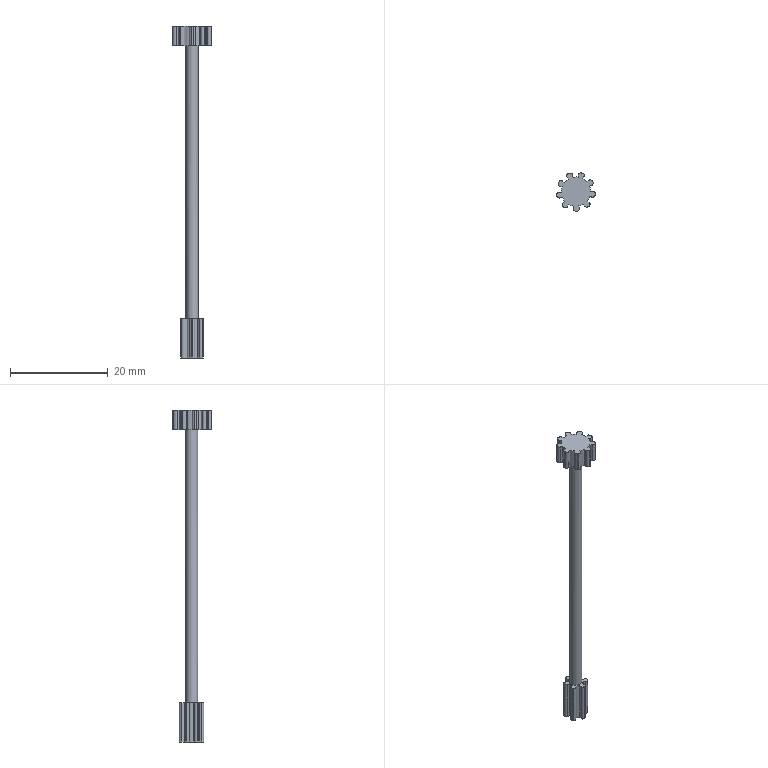Component | NX | LEADSCREW | 1 solid | 97 faces | volume 511 mm3 | cylinder 62 | plane 35 | commonest cylinder face diameters 1 x18 0.8 x12 8 x9 6 x9 5 x6 3 x6 2.5 x1 2.2 x1